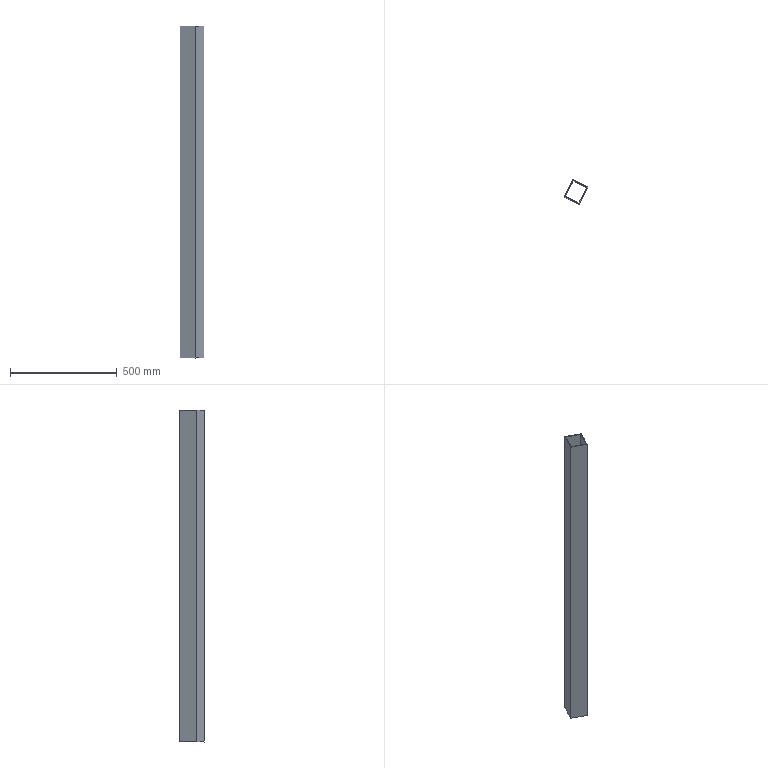Component | SolidWorks | Part10-1 | 1 solid | 10 faces | box 112.05 x 116.45 x 1554 mm | volume 2013984 mm3 | plane 10
build123d program:
from build123d import *

# Parameters (mm, degrees)
SKETCH1_W           = 1554
SKETCH1_H           = 90
BOSS_EXTRUDE1_DEPTH = 80
SHELL1_T            = -4


with BuildPart() as part:
    # Sketch1 → Boss-Extrude1 (new body)
    with BuildSketch(Plane.XY):
        with Locations((715.859, 21.801)):
            Rectangle(SKETCH1_W, SKETCH1_H)
    extrude(amount=BOSS_EXTRUDE1_DEPTH)

    # Shell1
    shell1_openings = [part.faces().sort_by_distance(p)[0] for p in [
        (1492.859, 21.801, 40),
        (-61.141, 21.801, 40),
    ]]
    offset(amount=SHELL1_T, openings=shell1_openings, kind=Kind.INTERSECTION)


solid = part.part

# Placed as in the assembly
solid = solid.moved(Location((300.189, -1142.672, 1097.113), (-90, -63.121, -90)))
STEP:
#1=COLOUR_RGB('',0.7922,0.8196,0.9333);
#2=FILL_AREA_STYLE_COLOUR('',#1);
#3=FILL_AREA_STYLE('',(#2));
#4=SURFACE_STYLE_FILL_AREA(#3);
#5=SURFACE_SIDE_STYLE('',(#4));
#6=SURFACE_STYLE_USAGE(.BOTH.,#5);
#7=PRESENTATION_STYLE_ASSIGNMENT((#6));
#8=CARTESIAN_POINT('',(13.007,-42.641,40.786));
#9=VERTEX_POINT('',#8);
#10=CARTESIAN_POINT('',(11.406,-45.802,40.786));
#11=VERTEX_POINT('',#10);
#12=CARTESIAN_POINT('',(13.007,-42.641,40.786));
#13=DIRECTION('',(-0.4521,-0.892,-0.));
#14=VECTOR('',#13,39.37);
#15=LINE('',#12,#14);
#16=EDGE_CURVE('',#9,#11,#15,.T.);
#17=ORIENTED_EDGE('',*,*,#16,.T.);
#18=CARTESIAN_POINT('',(8.596,-44.378,40.786));
#19=VERTEX_POINT('',#18);
#20=CARTESIAN_POINT('',(8.596,-44.378,40.786));
#21=DIRECTION('',(0.892,-0.4521,-0.));
#22=VECTOR('',#21,39.37);
#23=LINE('',#20,#22);
#24=EDGE_CURVE('',#19,#11,#23,.T.);
#25=ORIENTED_EDGE('',*,*,#24,.F.);
#26=CARTESIAN_POINT('',(10.198,-41.217,40.786));
#27=VERTEX_POINT('',#26);
#28=CARTESIAN_POINT('',(10.198,-41.217,40.786));
#29=DIRECTION('',(-0.4521,-0.892,-0.));
#30=VECTOR('',#29,39.37);
#31=LINE('',#28,#30);
#32=EDGE_CURVE('',#27,#19,#31,.T.);
#33=ORIENTED_EDGE('',*,*,#32,.F.);
#34=CARTESIAN_POINT('',(10.198,-41.217,40.786));
#35=DIRECTION('',(0.892,-0.4521,-0.));
#36=VECTOR('',#35,39.37);
#37=LINE('',#34,#36);
#38=EDGE_CURVE('',#27,#9,#37,.T.);
#39=ORIENTED_EDGE('',*,*,#38,.T.);
#40=EDGE_LOOP('',(#17,#25,#33,#39));
#41=FACE_OUTER_BOUND('',#40,.T.);
#42=CARTESIAN_POINT('',(12.796,-42.71,40.786));
#43=VERTEX_POINT('',#42);
#44=CARTESIAN_POINT('',(11.336,-45.59,40.786));
#45=VERTEX_POINT('',#44);
#46=CARTESIAN_POINT('',(12.867,-42.57,40.786));
#47=DIRECTION('',(-0.4521,-0.892,-0.));
#48=VECTOR('',#47,39.37);
#49=LINE('',#46,#48);
#50=EDGE_CURVE('',#43,#45,#49,.T.);
#51=ORIENTED_EDGE('',*,*,#50,.F.);
#52=CARTESIAN_POINT('',(10.267,-41.429,40.786));
#53=VERTEX_POINT('',#52);
#54=CARTESIAN_POINT('',(10.127,-41.358,40.786));
#55=DIRECTION('',(0.892,-0.4521,-0.));
#56=VECTOR('',#55,39.37);
#57=LINE('',#54,#56);
#58=EDGE_CURVE('',#53,#43,#57,.T.);
#59=ORIENTED_EDGE('',*,*,#58,.F.);
#60=CARTESIAN_POINT('',(8.808,-44.309,40.786));
#61=VERTEX_POINT('',#60);
#62=CARTESIAN_POINT('',(10.339,-41.288,40.786));
#63=DIRECTION('',(-0.4521,-0.892,-0.));
#64=VECTOR('',#63,39.37);
#65=LINE('',#62,#64);
#66=EDGE_CURVE('',#53,#61,#65,.T.);
#67=ORIENTED_EDGE('',*,*,#66,.T.);
#68=CARTESIAN_POINT('',(8.667,-44.237,40.786));
#69=DIRECTION('',(0.892,-0.4521,-0.));
#70=VECTOR('',#69,39.37);
#71=LINE('',#68,#70);
#72=EDGE_CURVE('',#61,#45,#71,.T.);
#73=ORIENTED_EDGE('',*,*,#72,.T.);
#74=EDGE_LOOP('',(#51,#59,#67,#73));
#75=FACE_BOUND('',#74,.T.);
#76=CARTESIAN_POINT('',(10.198,-41.217,40.786));
#77=DIRECTION('',(-0.,-0.,1.));
#78=DIRECTION('',(0.4521,0.892,0.));
#79=AXIS2_PLACEMENT_3D('',#76,#77,#78);
#80=PLANE('',#79);
#81=ADVANCED_FACE('',(#41,#75),#80,.F.);
#82=CARTESIAN_POINT('',(11.406,-45.802,101.967));
#83=VERTEX_POINT('',#82);
#84=CARTESIAN_POINT('',(13.007,-42.641,101.967));
#85=VERTEX_POINT('',#84);
#86=CARTESIAN_POINT('',(13.007,-42.641,101.967));
#87=DIRECTION('',(0.4521,0.892,0.));
#88=VECTOR('',#87,39.37);
#89=LINE('',#86,#88);
#90=EDGE_CURVE('',#83,#85,#89,.T.);
#91=ORIENTED_EDGE('',*,*,#90,.T.);
#92=CARTESIAN_POINT('',(10.198,-41.217,101.967));
#93=VERTEX_POINT('',#92);
#94=CARTESIAN_POINT('',(10.198,-41.217,101.967));
#95=DIRECTION('',(0.892,-0.4521,-0.));
#96=VECTOR('',#95,39.37);
#97=LINE('',#94,#96);
#98=EDGE_CURVE('',#93,#85,#97,.T.);
#99=ORIENTED_EDGE('',*,*,#98,.F.);
#100=CARTESIAN_POINT('',(8.596,-44.378,101.967));
#101=VERTEX_POINT('',#100);
#102=CARTESIAN_POINT('',(10.198,-41.217,101.967));
#103=DIRECTION('',(0.4521,0.892,0.));
#104=VECTOR('',#103,39.37);
#105=LINE('',#102,#104);
#106=EDGE_CURVE('',#101,#93,#105,.T.);
#107=ORIENTED_EDGE('',*,*,#106,.F.);
#108=CARTESIAN_POINT('',(8.596,-44.378,101.967));
#109=DIRECTION('',(0.892,-0.4521,-0.));
#110=VECTOR('',#109,39.37);
#111=LINE('',#108,#110);
#112=EDGE_CURVE('',#101,#83,#111,.T.);
#113=ORIENTED_EDGE('',*,*,#112,.T.);
#114=EDGE_LOOP('',(#91,#99,#107,#113));
#115=FACE_OUTER_BOUND('',#114,.T.);
#116=CARTESIAN_POINT('',(11.336,-45.59,101.967));
#117=VERTEX_POINT('',#116);
#118=CARTESIAN_POINT('',(12.796,-42.71,101.967));
#119=VERTEX_POINT('',#118);
#120=CARTESIAN_POINT('',(12.867,-42.57,101.967));
#121=DIRECTION('',(0.4521,0.892,0.));
#122=VECTOR('',#121,39.37);
#123=LINE('',#120,#122);
#124=EDGE_CURVE('',#117,#119,#123,.T.);
#125=ORIENTED_EDGE('',*,*,#124,.F.);
#126=CARTESIAN_POINT('',(8.808,-44.309,101.967));
#127=VERTEX_POINT('',#126);
#128=CARTESIAN_POINT('',(8.667,-44.237,101.967));
#129=DIRECTION('',(0.892,-0.4521,-0.));
#130=VECTOR('',#129,39.37);
#131=LINE('',#128,#130);
#132=EDGE_CURVE('',#127,#117,#131,.T.);
#133=ORIENTED_EDGE('',*,*,#132,.F.);
#134=CARTESIAN_POINT('',(10.267,-41.429,101.967));
#135=VERTEX_POINT('',#134);
#136=CARTESIAN_POINT('',(10.339,-41.288,101.967));
#137=DIRECTION('',(0.4521,0.892,0.));
#138=VECTOR('',#137,39.37);
#139=LINE('',#136,#138);
#140=EDGE_CURVE('',#127,#135,#139,.T.);
#141=ORIENTED_EDGE('',*,*,#140,.T.);
#142=CARTESIAN_POINT('',(10.127,-41.358,101.967));
#143=DIRECTION('',(0.892,-0.4521,-0.));
#144=VECTOR('',#143,39.37);
#145=LINE('',#142,#144);
#146=EDGE_CURVE('',#135,#119,#145,.T.);
#147=ORIENTED_EDGE('',*,*,#146,.T.);
#148=EDGE_LOOP('',(#125,#133,#141,#147));
#149=FACE_BOUND('',#148,.T.);
#150=CARTESIAN_POINT('',(10.198,-41.217,101.967));
#151=DIRECTION('',(0.,0.,-1.));
#152=DIRECTION('',(-0.892,0.4521,0.));
#153=AXIS2_PLACEMENT_3D('',#150,#151,#152);
#154=PLANE('',#153);
#155=ADVANCED_FACE('',(#115,#149),#154,.F.);
#156=CARTESIAN_POINT('',(11.406,-45.802,40.786));
#157=DIRECTION('',(-0.,-0.,1.));
#158=VECTOR('',#157,39.37);
#159=LINE('',#156,#158);
#160=EDGE_CURVE('',#11,#83,#159,.T.);
#161=ORIENTED_EDGE('',*,*,#160,.T.);
#162=ORIENTED_EDGE('',*,*,#112,.F.);
#163=CARTESIAN_POINT('',(8.596,-44.378,40.786));
#164=DIRECTION('',(-0.,-0.,1.));
#165=VECTOR('',#164,39.37);
#166=LINE('',#163,#165);
#167=EDGE_CURVE('',#19,#101,#166,.T.);
#168=ORIENTED_EDGE('',*,*,#167,.F.);
#169=ORIENTED_EDGE('',*,*,#24,.T.);
#170=EDGE_LOOP('',(#161,#162,#168,#169));
#171=FACE_OUTER_BOUND('',#170,.T.);
#172=CARTESIAN_POINT('',(8.596,-44.378,40.786));
#173=DIRECTION('',(0.4521,0.892,0.));
#174=DIRECTION('',(-0.892,0.4521,0.));
#175=AXIS2_PLACEMENT_3D('',#172,#173,#174);
#176=PLANE('',#175);
#177=ADVANCED_FACE('',(#171),#176,.F.);
#178=CARTESIAN_POINT('',(13.007,-42.641,40.786));
#179=DIRECTION('',(0.,0.,-1.));
#180=VECTOR('',#179,39.37);
#181=LINE('',#178,#180);
#182=EDGE_CURVE('',#85,#9,#181,.T.);
#183=ORIENTED_EDGE('',*,*,#182,.T.);
#184=ORIENTED_EDGE('',*,*,#38,.F.);
#185=CARTESIAN_POINT('',(10.198,-41.217,40.786));
#186=DIRECTION('',(0.,0.,-1.));
#187=VECTOR('',#186,39.37);
#188=LINE('',#185,#187);
#189=EDGE_CURVE('',#93,#27,#188,.T.);
#190=ORIENTED_EDGE('',*,*,#189,.F.);
#191=ORIENTED_EDGE('',*,*,#98,.T.);
#192=EDGE_LOOP('',(#183,#184,#190,#191));
#193=FACE_OUTER_BOUND('',#192,.T.);
#194=CARTESIAN_POINT('',(10.198,-41.217,40.786));
#195=DIRECTION('',(-0.4521,-0.892,-0.));
#196=DIRECTION('',(0.892,-0.4521,-0.));
#197=AXIS2_PLACEMENT_3D('',#194,#195,#196);
#198=PLANE('',#197);
#199=ADVANCED_FACE('',(#193),#198,.F.);
#200=ORIENTED_EDGE('',*,*,#32,.T.);
#201=ORIENTED_EDGE('',*,*,#167,.T.);
#202=ORIENTED_EDGE('',*,*,#106,.T.);
#203=ORIENTED_EDGE('',*,*,#189,.T.);
#204=EDGE_LOOP('',(#200,#201,#202,#203));
#205=FACE_OUTER_BOUND('',#204,.T.);
#206=CARTESIAN_POINT('',(9.009,-43.563,43.193));
#207=DIRECTION('',(-0.892,0.4521,0.));
#208=DIRECTION('',(-0.,-0.,1.));
#209=AXIS2_PLACEMENT_3D('',#206,#207,#208);
#210=PLANE('',#209);
#211=ADVANCED_FACE('',(#205),#210,.T.);
#212=ORIENTED_EDGE('',*,*,#16,.F.);
#213=ORIENTED_EDGE('',*,*,#182,.F.);
#214=ORIENTED_EDGE('',*,*,#90,.F.);
#215=ORIENTED_EDGE('',*,*,#160,.F.);
#216=EDGE_LOOP('',(#212,#213,#214,#215));
#217=FACE_OUTER_BOUND('',#216,.T.);
#218=CARTESIAN_POINT('',(11.818,-44.987,43.193));
#219=DIRECTION('',(-0.892,0.4521,0.));
#220=DIRECTION('',(-0.,-0.,1.));
#221=AXIS2_PLACEMENT_3D('',#218,#219,#220);
#222=PLANE('',#221);
#223=ADVANCED_FACE('',(#217),#222,.F.);
#224=CARTESIAN_POINT('',(11.336,-45.59,40.786));
#225=DIRECTION('',(-0.,-0.,1.));
#226=VECTOR('',#225,39.37);
#227=LINE('',#224,#226);
#228=EDGE_CURVE('',#45,#117,#227,.T.);
#229=ORIENTED_EDGE('',*,*,#228,.F.);
#230=ORIENTED_EDGE('',*,*,#72,.F.);
#231=CARTESIAN_POINT('',(8.808,-44.309,40.786));
#232=DIRECTION('',(-0.,-0.,1.));
#233=VECTOR('',#232,39.37);
#234=LINE('',#231,#233);
#235=EDGE_CURVE('',#61,#127,#234,.T.);
#236=ORIENTED_EDGE('',*,*,#235,.T.);
#237=ORIENTED_EDGE('',*,*,#132,.T.);
#238=EDGE_LOOP('',(#229,#230,#236,#237));
#239=FACE_OUTER_BOUND('',#238,.T.);
#240=CARTESIAN_POINT('',(8.667,-44.237,40.786));
#241=DIRECTION('',(0.4521,0.892,0.));
#242=DIRECTION('',(-0.892,0.4521,0.));
#243=AXIS2_PLACEMENT_3D('',#240,#241,#242);
#244=PLANE('',#243);
#245=ADVANCED_FACE('',(#239),#244,.T.);
#246=CARTESIAN_POINT('',(12.796,-42.71,40.786));
#247=DIRECTION('',(0.,0.,-1.));
#248=VECTOR('',#247,39.37);
#249=LINE('',#246,#248);
#250=EDGE_CURVE('',#119,#43,#249,.T.);
#251=ORIENTED_EDGE('',*,*,#250,.F.);
#252=ORIENTED_EDGE('',*,*,#146,.F.);
#253=CARTESIAN_POINT('',(10.267,-41.429,40.786));
#254=DIRECTION('',(0.,0.,-1.));
#255=VECTOR('',#254,39.37);
#256=LINE('',#253,#255);
#257=EDGE_CURVE('',#135,#53,#256,.T.);
#258=ORIENTED_EDGE('',*,*,#257,.T.);
#259=ORIENTED_EDGE('',*,*,#58,.T.);
#260=EDGE_LOOP('',(#251,#252,#258,#259));
#261=FACE_OUTER_BOUND('',#260,.T.);
#262=CARTESIAN_POINT('',(10.127,-41.358,40.786));
#263=DIRECTION('',(-0.4521,-0.892,-0.));
#264=DIRECTION('',(0.892,-0.4521,-0.));
#265=AXIS2_PLACEMENT_3D('',#262,#263,#264);
#266=PLANE('',#265);
#267=ADVANCED_FACE('',(#261),#266,.T.);
#268=ORIENTED_EDGE('',*,*,#66,.F.);
#269=ORIENTED_EDGE('',*,*,#257,.F.);
#270=ORIENTED_EDGE('',*,*,#140,.F.);
#271=ORIENTED_EDGE('',*,*,#235,.F.);
#272=EDGE_LOOP('',(#268,#269,#270,#271));
#273=FACE_OUTER_BOUND('',#272,.T.);
#274=CARTESIAN_POINT('',(9.15,-43.634,43.193));
#275=DIRECTION('',(-0.892,0.4521,0.));
#276=DIRECTION('',(-0.,-0.,1.));
#277=AXIS2_PLACEMENT_3D('',#274,#275,#276);
#278=PLANE('',#277);
#279=ADVANCED_FACE('',(#273),#278,.F.);
#280=ORIENTED_EDGE('',*,*,#50,.T.);
#281=ORIENTED_EDGE('',*,*,#228,.T.);
#282=ORIENTED_EDGE('',*,*,#124,.T.);
#283=ORIENTED_EDGE('',*,*,#250,.T.);
#284=EDGE_LOOP('',(#280,#281,#282,#283));
#285=FACE_OUTER_BOUND('',#284,.T.);
#286=CARTESIAN_POINT('',(11.678,-44.916,43.193));
#287=DIRECTION('',(-0.892,0.4521,0.));
#288=DIRECTION('',(-0.,-0.,1.));
#289=AXIS2_PLACEMENT_3D('',#286,#287,#288);
#290=PLANE('',#289);
#291=ADVANCED_FACE('',(#285),#290,.T.);
#292=CLOSED_SHELL('',(#81,#155,#177,#199,#211,#223,#245,#267,#279,#291));
#293=MANIFOLD_SOLID_BREP('',#292);
#294=STYLED_ITEM('',(#7),#293);
#295=(LENGTH_UNIT()NAMED_UNIT(*)SI_UNIT($,.METRE.));
#296=LENGTH_MEASURE_WITH_UNIT(LENGTH_MEASURE(0.0254),#295);
#297=DIMENSIONAL_EXPONENTS(1.,0.,0.,0.,0.,0.,0.);
#298=(CONVERSION_BASED_UNIT('',#296)LENGTH_UNIT()NAMED_UNIT(#297));
#299=UNCERTAINTY_MEASURE_WITH_UNIT(LENGTH_MEASURE(0.00001),#298,'','');
#300=(NAMED_UNIT(*)PLANE_ANGLE_UNIT()SI_UNIT($,.RADIAN.));
#301=(NAMED_UNIT(*)SI_UNIT($,.STERADIAN.)SOLID_ANGLE_UNIT());
#302=(GEOMETRIC_REPRESENTATION_CONTEXT(3)GLOBAL_UNCERTAINTY_ASSIGNED_CONTEXT((#299))GLOBAL_UNIT_ASSIGNED_CONTEXT((#298,#300,#301))REPRESENTATION_CONTEXT('',''));
#303=MECHANICAL_DESIGN_GEOMETRIC_PRESENTATION_REPRESENTATION('',(#294),#302);
#304=CARTESIAN_POINT('',(0.,0.,0.));
#305=DIRECTION('',(0.,0.,1.));
#306=DIRECTION('',(1.,0.,0.));
#307=AXIS2_PLACEMENT_3D('',#304,#305,#306);
#308=(LENGTH_UNIT()NAMED_UNIT(*)SI_UNIT($,.METRE.));
#309=LENGTH_MEASURE_WITH_UNIT(LENGTH_MEASURE(0.0254),#308);
#310=DIMENSIONAL_EXPONENTS(1.,0.,0.,0.,0.,0.,0.);
#311=(CONVERSION_BASED_UNIT('',#309)LENGTH_UNIT()NAMED_UNIT(#310));
#312=UNCERTAINTY_MEASURE_WITH_UNIT(LENGTH_MEASURE(0.00001),#311,'','');
#313=(NAMED_UNIT(*)PLANE_ANGLE_UNIT()SI_UNIT($,.RADIAN.));
#314=(NAMED_UNIT(*)SI_UNIT($,.STERADIAN.)SOLID_ANGLE_UNIT());
#315=(GEOMETRIC_REPRESENTATION_CONTEXT(3)GLOBAL_UNCERTAINTY_ASSIGNED_CONTEXT((#312))GLOBAL_UNIT_ASSIGNED_CONTEXT((#311,#313,#314))REPRESENTATION_CONTEXT('',''));
#316=ADVANCED_BREP_SHAPE_REPRESENTATION('',(#293,#307),#315);
#317=PRESENTATION_LAYER_ASSIGNMENT('','',(#294));